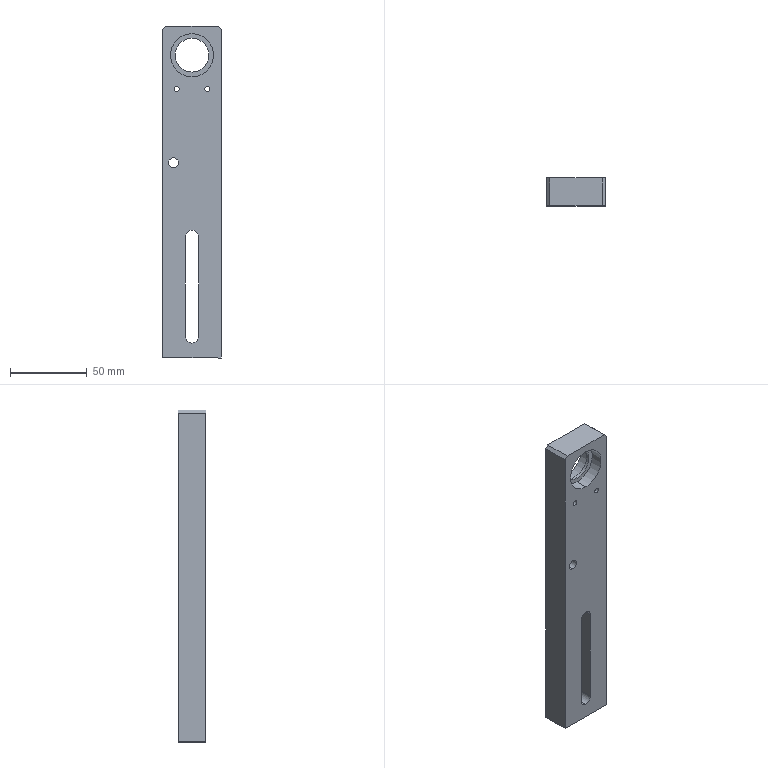Component | SolidWorks | FixedBlock2-1 | 1 solid | 30 faces | box 38 x 18 x 216 mm | volume 124786 mm3 | cylinder 17 | plane 13 | commonest cylinder face diameters 3.3 x4 28 x4 8.5 x3 11 x2 6.5 x2 22 x2
build123d program:
from build123d import *

# Parameters (mm, degrees)
SKETCH1_W                                          = 216
SKETCH1_H                                          = 38
BOSS_EXTRUDE1_DEPTH                                = 18
SKETCH3_R                                          = 11
CUT_EXTRUDE1_DEPTH                                 = 18
SKETCH4_R                                          = 14
CUT_EXTRUDE2_DEPTH                                 = 8
CUT_EXTRUDE3_START                                 = -8
SKETCH5_R                                          = 14
CUT_EXTRUDE3_DEPTH                                 = 8
CUT_EXTRUDE4_DEPTH                                 = 73
CHAMFER1_SIZE                                      = 2
M4_TAPPED_HOLE1_D                                  = 3.3
HOLE_SIZE_ACCORDING_TO_TYPE_1_OF_HEXAG_D           = 6.5
HOLE_SIZE_ACCORDING_TO_TYPE_1_OF_HEXAG_CBORE_D     = 11
HOLE_SIZE_ACCORDING_TO_TYPE_1_OF_HEXAG_CBORE_DEPTH = 6.5


with BuildPart() as part:
    # Sketch1 → Boss-Extrude1 (new body)
    with BuildSketch(Plane.XY):
        Rectangle(SKETCH1_W, SKETCH1_H)
    extrude(amount=BOSS_EXTRUDE1_DEPTH)

    # Sketch3 → Cut-Extrude1 (cut)
    with BuildSketch(Plane.XY.offset(18)):
        with Locations((89, 0)):
            Circle(SKETCH3_R)
    extrude(amount=-CUT_EXTRUDE1_DEPTH, mode=Mode.SUBTRACT)

    # Sketch4 → Cut-Extrude2 (cut)
    with BuildSketch(Plane.XY.offset(18)):
        with Locations((89, 0)):
            Circle(SKETCH4_R)
    extrude(amount=-CUT_EXTRUDE2_DEPTH, mode=Mode.SUBTRACT)

    # Sketch5 → Cut-Extrude3 (cut)
    with BuildSketch(Plane(origin=(0, 0, 0), x_dir=(-1, 0, 0), z_dir=(0, 0, -1)).offset(CUT_EXTRUDE3_START)):
        with Locations(Location((-89, 0, 0), (0, 0, 180))):
            Circle(SKETCH5_R)
    extrude(amount=CUT_EXTRUDE3_DEPTH, mode=Mode.SUBTRACT)

    # Sketch6 → Cut-Extrude4 (cut)
    with BuildSketch(Plane(origin=(0, 0, 0), x_dir=(-1, 0, 0), z_dir=(0, 0, -1))):
        with BuildLine():
            Line((29, 4.25), (94, 4.25))
            ThreePointArc((94, 4.25), (98.25, 0), (94, -4.25))
            Line((94, -4.25), (29, -4.25))
            ThreePointArc((29, -4.25), (24.75, 0), (29, 4.25))
        make_face()
    extrude(amount=-CUT_EXTRUDE4_DEPTH, mode=Mode.SUBTRACT)

    # Chamfer1
    chamfer1_edges = [part.edges().sort_by_distance(p)[0] for p in [
        (108, -19, 9),
        (108, 19, 9),
    ]]
    chamfer(chamfer1_edges, length=CHAMFER1_SIZE)

    # M4 Tapped Hole1 (through all)
    with Locations(Plane(origin=(67, -10, 0), x_dir=(-1, 0, 0), z_dir=(0, 0, -1))):
        with Locations((0, 0), (0, 20)):
            Hole(M4_TAPPED_HOLE1_D / 2)

    # Hole Size _according to_ Type 1 of Hexag (through all)
    with Locations(Plane(origin=(19, -12, 18), x_dir=(1, 0, 0), z_dir=(0, 0, 1))):
        with Locations((0, 0)):
            CounterBoreHole(HOLE_SIZE_ACCORDING_TO_TYPE_1_OF_HEXAG_D / 2, HOLE_SIZE_ACCORDING_TO_TYPE_1_OF_HEXAG_CBORE_D / 2, HOLE_SIZE_ACCORDING_TO_TYPE_1_OF_HEXAG_CBORE_DEPTH)


solid = part.part

# Placed as in the assembly
solid = solid.moved(Location((-48.547, -21.54, 239), (-90, 0, -90)))
STEP:
#1=CARTESIAN_POINT('',(-2.384,-0.3953,9.941));
#2=VERTEX_POINT('',#1);
#3=CARTESIAN_POINT('',(-2.384,-0.3953,10.374));
#4=VERTEX_POINT('',#3);
#5=CARTESIAN_POINT('',(-2.384,-0.3953,10.157));
#6=DIRECTION('',(-0.,1.,-0.));
#7=DIRECTION('',(0.,0.,1.));
#8=AXIS2_PLACEMENT_3D('',#5,#6,#7);
#9=CIRCLE('',#8,0.2165);
#10=EDGE_CURVE('',#2,#4,#9,.T.);
#11=ORIENTED_EDGE('',*,*,#10,.F.);
#12=CARTESIAN_POINT('',(-2.384,-0.1394,9.941));
#13=VERTEX_POINT('',#12);
#14=CARTESIAN_POINT('',(-2.384,-0.1394,9.941));
#15=DIRECTION('',(-0.,1.,-0.));
#16=VECTOR('',#15,39.37);
#17=LINE('',#14,#16);
#18=EDGE_CURVE('',#2,#13,#17,.T.);
#19=ORIENTED_EDGE('',*,*,#18,.T.);
#20=CARTESIAN_POINT('',(-2.384,-0.1394,10.374));
#21=VERTEX_POINT('',#20);
#22=CARTESIAN_POINT('',(-2.384,-0.1394,10.157));
#23=DIRECTION('',(-0.,1.,-0.));
#24=DIRECTION('',(0.,0.,1.));
#25=AXIS2_PLACEMENT_3D('',#22,#23,#24);
#26=CIRCLE('',#25,0.2165);
#27=EDGE_CURVE('',#13,#21,#26,.T.);
#28=ORIENTED_EDGE('',*,*,#27,.T.);
#29=CARTESIAN_POINT('',(-2.384,-0.1394,10.374));
#30=DIRECTION('',(-0.,1.,-0.));
#31=VECTOR('',#30,39.37);
#32=LINE('',#29,#31);
#33=EDGE_CURVE('',#4,#21,#32,.T.);
#34=ORIENTED_EDGE('',*,*,#33,.F.);
#35=EDGE_LOOP('',(#11,#19,#28,#34));
#36=FACE_OUTER_BOUND('',#35,.T.);
#37=CARTESIAN_POINT('',(-2.384,-0.1394,10.157));
#38=DIRECTION('',(-0.,1.,-0.));
#39=DIRECTION('',(0.,0.,1.));
#40=AXIS2_PLACEMENT_3D('',#37,#38,#39);
#41=CYLINDRICAL_SURFACE('',#40,0.2165);
#42=ADVANCED_FACE('',(#36),#41,.F.);
#43=CARTESIAN_POINT('',(-2.384,-0.848,10.285));
#44=VERTEX_POINT('',#43);
#45=CARTESIAN_POINT('',(-2.384,-0.848,10.03));
#46=VERTEX_POINT('',#45);
#47=CARTESIAN_POINT('',(-2.384,-0.848,10.157));
#48=DIRECTION('',(0.,-1.,0.));
#49=DIRECTION('',(-0.,0.,-1.));
#50=AXIS2_PLACEMENT_3D('',#47,#48,#49);
#51=CIRCLE('',#50,0.128);
#52=EDGE_CURVE('',#44,#46,#51,.T.);
#53=ORIENTED_EDGE('',*,*,#52,.T.);
#54=CARTESIAN_POINT('',(-2.384,-0.3953,10.03));
#55=VERTEX_POINT('',#54);
#56=CARTESIAN_POINT('',(-2.384,-0.1394,10.03));
#57=DIRECTION('',(-0.,1.,-0.));
#58=VECTOR('',#57,39.37);
#59=LINE('',#56,#58);
#60=EDGE_CURVE('',#46,#55,#59,.T.);
#61=ORIENTED_EDGE('',*,*,#60,.T.);
#62=CARTESIAN_POINT('',(-2.384,-0.3953,10.285));
#63=VERTEX_POINT('',#62);
#64=CARTESIAN_POINT('',(-2.384,-0.3953,10.157));
#65=DIRECTION('',(-0.,1.,-0.));
#66=DIRECTION('',(0.,0.,1.));
#67=AXIS2_PLACEMENT_3D('',#64,#65,#66);
#68=CIRCLE('',#67,0.128);
#69=EDGE_CURVE('',#55,#63,#68,.T.);
#70=ORIENTED_EDGE('',*,*,#69,.T.);
#71=CARTESIAN_POINT('',(-2.384,-0.1394,10.285));
#72=DIRECTION('',(-0.,1.,-0.));
#73=VECTOR('',#72,39.37);
#74=LINE('',#71,#73);
#75=EDGE_CURVE('',#44,#63,#74,.T.);
#76=ORIENTED_EDGE('',*,*,#75,.F.);
#77=EDGE_LOOP('',(#53,#61,#70,#76));
#78=FACE_OUTER_BOUND('',#77,.T.);
#79=CARTESIAN_POINT('',(-2.384,-0.1394,10.157));
#80=DIRECTION('',(-0.,1.,-0.));
#81=DIRECTION('',(0.,0.,1.));
#82=AXIS2_PLACEMENT_3D('',#79,#80,#81);
#83=CYLINDRICAL_SURFACE('',#82,0.128);
#84=ADVANCED_FACE('',(#78),#83,.F.);
#85=CARTESIAN_POINT('',(-2.305,-0.1394,12.112));
#86=VERTEX_POINT('',#85);
#87=CARTESIAN_POINT('',(-2.305,-0.1394,11.982));
#88=VERTEX_POINT('',#87);
#89=CARTESIAN_POINT('',(-2.305,-0.1394,12.047));
#90=DIRECTION('',(0.,-1.,0.));
#91=DIRECTION('',(-0.,0.,-1.));
#92=AXIS2_PLACEMENT_3D('',#89,#90,#91);
#93=CIRCLE('',#92,0.06496);
#94=EDGE_CURVE('',#86,#88,#93,.T.);
#95=ORIENTED_EDGE('',*,*,#94,.F.);
#96=CARTESIAN_POINT('',(-2.305,-0.848,12.112));
#97=VERTEX_POINT('',#96);
#98=CARTESIAN_POINT('',(-2.305,-0.848,12.112));
#99=DIRECTION('',(0.,-1.,0.));
#100=VECTOR('',#99,39.37);
#101=LINE('',#98,#100);
#102=EDGE_CURVE('',#86,#97,#101,.T.);
#103=ORIENTED_EDGE('',*,*,#102,.T.);
#104=CARTESIAN_POINT('',(-2.305,-0.848,11.982));
#105=VERTEX_POINT('',#104);
#106=CARTESIAN_POINT('',(-2.305,-0.848,12.047));
#107=DIRECTION('',(0.,-1.,0.));
#108=DIRECTION('',(-0.,0.,-1.));
#109=AXIS2_PLACEMENT_3D('',#106,#107,#108);
#110=CIRCLE('',#109,0.06496);
#111=EDGE_CURVE('',#97,#105,#110,.T.);
#112=ORIENTED_EDGE('',*,*,#111,.T.);
#113=CARTESIAN_POINT('',(-2.305,-0.848,11.982));
#114=DIRECTION('',(0.,-1.,0.));
#115=VECTOR('',#114,39.37);
#116=LINE('',#113,#115);
#117=EDGE_CURVE('',#88,#105,#116,.T.);
#118=ORIENTED_EDGE('',*,*,#117,.F.);
#119=EDGE_LOOP('',(#95,#103,#112,#118));
#120=FACE_OUTER_BOUND('',#119,.T.);
#121=CARTESIAN_POINT('',(-2.305,-0.848,12.047));
#122=DIRECTION('',(0.,-1.,0.));
#123=DIRECTION('',(-0.,0.,-1.));
#124=AXIS2_PLACEMENT_3D('',#121,#122,#123);
#125=CYLINDRICAL_SURFACE('',#124,0.06496);
#126=ADVANCED_FACE('',(#120),#125,.F.);
#127=CARTESIAN_POINT('',(-1.518,-0.1394,12.112));
#128=VERTEX_POINT('',#127);
#129=CARTESIAN_POINT('',(-1.518,-0.1394,11.982));
#130=VERTEX_POINT('',#129);
#131=CARTESIAN_POINT('',(-1.518,-0.1394,12.047));
#132=DIRECTION('',(0.,-1.,0.));
#133=DIRECTION('',(-0.,0.,-1.));
#134=AXIS2_PLACEMENT_3D('',#131,#132,#133);
#135=CIRCLE('',#134,0.06496);
#136=EDGE_CURVE('',#128,#130,#135,.T.);
#137=ORIENTED_EDGE('',*,*,#136,.F.);
#138=CARTESIAN_POINT('',(-1.518,-0.848,12.112));
#139=VERTEX_POINT('',#138);
#140=CARTESIAN_POINT('',(-1.518,-0.848,12.112));
#141=DIRECTION('',(0.,-1.,0.));
#142=VECTOR('',#141,39.37);
#143=LINE('',#140,#142);
#144=EDGE_CURVE('',#128,#139,#143,.T.);
#145=ORIENTED_EDGE('',*,*,#144,.T.);
#146=CARTESIAN_POINT('',(-1.518,-0.848,11.982));
#147=VERTEX_POINT('',#146);
#148=CARTESIAN_POINT('',(-1.518,-0.848,12.047));
#149=DIRECTION('',(0.,-1.,0.));
#150=DIRECTION('',(-0.,0.,-1.));
#151=AXIS2_PLACEMENT_3D('',#148,#149,#150);
#152=CIRCLE('',#151,0.06496);
#153=EDGE_CURVE('',#139,#147,#152,.T.);
#154=ORIENTED_EDGE('',*,*,#153,.T.);
#155=CARTESIAN_POINT('',(-1.518,-0.848,11.982));
#156=DIRECTION('',(0.,-1.,0.));
#157=VECTOR('',#156,39.37);
#158=LINE('',#155,#157);
#159=EDGE_CURVE('',#130,#147,#158,.T.);
#160=ORIENTED_EDGE('',*,*,#159,.F.);
#161=EDGE_LOOP('',(#137,#145,#154,#160));
#162=FACE_OUTER_BOUND('',#161,.T.);
#163=CARTESIAN_POINT('',(-1.518,-0.848,12.047));
#164=DIRECTION('',(0.,-1.,0.));
#165=DIRECTION('',(-0.,0.,-1.));
#166=AXIS2_PLACEMENT_3D('',#163,#164,#165);
#167=CYLINDRICAL_SURFACE('',#166,0.06496);
#168=ADVANCED_FACE('',(#162),#167,.F.);
#169=CARTESIAN_POINT('',(-1.911,-0.1394,5.541));
#170=VERTEX_POINT('',#169);
#171=CARTESIAN_POINT('',(-1.744,-0.1394,5.709));
#172=VERTEX_POINT('',#171);
#173=CARTESIAN_POINT('',(-1.911,-0.1394,5.709));
#174=DIRECTION('',(0.,-1.,0.));
#175=DIRECTION('',(-0.,0.,-1.));
#176=AXIS2_PLACEMENT_3D('',#173,#174,#175);
#177=CIRCLE('',#176,0.1673);
#178=EDGE_CURVE('',#170,#172,#177,.T.);
#179=ORIENTED_EDGE('',*,*,#178,.F.);
#180=CARTESIAN_POINT('',(-1.911,-0.848,5.541));
#181=VERTEX_POINT('',#180);
#182=CARTESIAN_POINT('',(-1.911,2.026,5.541));
#183=DIRECTION('',(0.,-1.,0.));
#184=VECTOR('',#183,39.37);
#185=LINE('',#182,#184);
#186=EDGE_CURVE('',#170,#181,#185,.T.);
#187=ORIENTED_EDGE('',*,*,#186,.T.);
#188=CARTESIAN_POINT('',(-1.744,-0.848,5.709));
#189=VERTEX_POINT('',#188);
#190=CARTESIAN_POINT('',(-1.911,-0.848,5.709));
#191=DIRECTION('',(0.,-1.,0.));
#192=DIRECTION('',(-0.,0.,-1.));
#193=AXIS2_PLACEMENT_3D('',#190,#191,#192);
#194=CIRCLE('',#193,0.1673);
#195=EDGE_CURVE('',#181,#189,#194,.T.);
#196=ORIENTED_EDGE('',*,*,#195,.T.);
#197=CARTESIAN_POINT('',(-1.744,2.026,5.709));
#198=DIRECTION('',(0.,-1.,0.));
#199=VECTOR('',#198,39.37);
#200=LINE('',#197,#199);
#201=EDGE_CURVE('',#172,#189,#200,.T.);
#202=ORIENTED_EDGE('',*,*,#201,.F.);
#203=EDGE_LOOP('',(#179,#187,#196,#202));
#204=FACE_OUTER_BOUND('',#203,.T.);
#205=CARTESIAN_POINT('',(-1.911,2.026,5.709));
#206=DIRECTION('',(0.,-1.,0.));
#207=DIRECTION('',(-0.,0.,-1.));
#208=AXIS2_PLACEMENT_3D('',#205,#206,#207);
#209=CYLINDRICAL_SURFACE('',#208,0.1673);
#210=ADVANCED_FACE('',(#204),#209,.F.);
#211=CARTESIAN_POINT('',(-1.911,-0.5331,13.465));
#212=VERTEX_POINT('',#211);
#213=CARTESIAN_POINT('',(-1.911,-0.5331,12.362));
#214=VERTEX_POINT('',#213);
#215=CARTESIAN_POINT('',(-1.911,-0.5331,12.913));
#216=DIRECTION('',(0.,-1.,0.));
#217=DIRECTION('',(-0.,0.,-1.));
#218=AXIS2_PLACEMENT_3D('',#215,#216,#217);
#219=CIRCLE('',#218,0.5512);
#220=EDGE_CURVE('',#212,#214,#219,.T.);
#221=ORIENTED_EDGE('',*,*,#220,.F.);
#222=CARTESIAN_POINT('',(-1.911,-0.848,13.465));
#223=VERTEX_POINT('',#222);
#224=CARTESIAN_POINT('',(-1.911,-0.5331,13.465));
#225=DIRECTION('',(0.,-1.,0.));
#226=VECTOR('',#225,39.37);
#227=LINE('',#224,#226);
#228=EDGE_CURVE('',#212,#223,#227,.T.);
#229=ORIENTED_EDGE('',*,*,#228,.T.);
#230=CARTESIAN_POINT('',(-1.911,-0.848,12.362));
#231=VERTEX_POINT('',#230);
#232=CARTESIAN_POINT('',(-1.911,-0.848,12.913));
#233=DIRECTION('',(0.,-1.,0.));
#234=DIRECTION('',(-0.,0.,-1.));
#235=AXIS2_PLACEMENT_3D('',#232,#233,#234);
#236=CIRCLE('',#235,0.5512);
#237=EDGE_CURVE('',#223,#231,#236,.T.);
#238=ORIENTED_EDGE('',*,*,#237,.T.);
#239=CARTESIAN_POINT('',(-1.911,-0.5331,12.362));
#240=DIRECTION('',(0.,-1.,0.));
#241=VECTOR('',#240,39.37);
#242=LINE('',#239,#241);
#243=EDGE_CURVE('',#214,#231,#242,.T.);
#244=ORIENTED_EDGE('',*,*,#243,.F.);
#245=EDGE_LOOP('',(#221,#229,#238,#244));
#246=FACE_OUTER_BOUND('',#245,.T.);
#247=CARTESIAN_POINT('',(-1.911,-0.5331,12.913));
#248=DIRECTION('',(0.,-1.,0.));
#249=DIRECTION('',(-0.,0.,-1.));
#250=AXIS2_PLACEMENT_3D('',#247,#248,#249);
#251=CYLINDRICAL_SURFACE('',#250,0.5512);
#252=ADVANCED_FACE('',(#246),#251,.F.);
#253=CARTESIAN_POINT('',(-1.911,-0.4543,12.362));
#254=VERTEX_POINT('',#253);
#255=CARTESIAN_POINT('',(-1.911,-0.4543,13.465));
#256=VERTEX_POINT('',#255);
#257=CARTESIAN_POINT('',(-1.911,-0.4543,12.913));
#258=DIRECTION('',(-0.,1.,-0.));
#259=DIRECTION('',(0.,0.,1.));
#260=AXIS2_PLACEMENT_3D('',#257,#258,#259);
#261=CIRCLE('',#260,0.5512);
#262=EDGE_CURVE('',#254,#256,#261,.T.);
#263=ORIENTED_EDGE('',*,*,#262,.F.);
#264=CARTESIAN_POINT('',(-1.911,-0.1394,12.362));
#265=VERTEX_POINT('',#264);
#266=CARTESIAN_POINT('',(-1.911,-0.4543,12.362));
#267=DIRECTION('',(-0.,1.,-0.));
#268=VECTOR('',#267,39.37);
#269=LINE('',#266,#268);
#270=EDGE_CURVE('',#254,#265,#269,.T.);
#271=ORIENTED_EDGE('',*,*,#270,.T.);
#272=CARTESIAN_POINT('',(-1.911,-0.1394,13.465));
#273=VERTEX_POINT('',#272);
#274=CARTESIAN_POINT('',(-1.911,-0.1394,12.913));
#275=DIRECTION('',(-0.,1.,-0.));
#276=DIRECTION('',(0.,0.,1.));
#277=AXIS2_PLACEMENT_3D('',#274,#275,#276);
#278=CIRCLE('',#277,0.5512);
#279=EDGE_CURVE('',#265,#273,#278,.T.);
#280=ORIENTED_EDGE('',*,*,#279,.T.);
#281=CARTESIAN_POINT('',(-1.911,-0.4543,13.465));
#282=DIRECTION('',(-0.,1.,-0.));
#283=VECTOR('',#282,39.37);
#284=LINE('',#281,#283);
#285=EDGE_CURVE('',#256,#273,#284,.T.);
#286=ORIENTED_EDGE('',*,*,#285,.F.);
#287=EDGE_LOOP('',(#263,#271,#280,#286));
#288=FACE_OUTER_BOUND('',#287,.T.);
#289=CARTESIAN_POINT('',(-1.911,-0.4543,12.913));
#290=DIRECTION('',(-0.,1.,-0.));
#291=DIRECTION('',(0.,0.,1.));
#292=AXIS2_PLACEMENT_3D('',#289,#290,#291);
#293=CYLINDRICAL_SURFACE('',#292,0.5512);
#294=ADVANCED_FACE('',(#288),#293,.F.);
#295=CARTESIAN_POINT('',(-1.911,-0.5331,12.48));
#296=VERTEX_POINT('',#295);
#297=CARTESIAN_POINT('',(-1.911,-0.5331,13.346));
#298=VERTEX_POINT('',#297);
#299=CARTESIAN_POINT('',(-1.911,-0.5331,12.913));
#300=DIRECTION('',(-0.,1.,-0.));
#301=DIRECTION('',(-0.,0.,-1.));
#302=AXIS2_PLACEMENT_3D('',#299,#300,#301);
#303=CIRCLE('',#302,0.4331);
#304=EDGE_CURVE('',#296,#298,#303,.T.);
#305=ORIENTED_EDGE('',*,*,#304,.F.);
#306=CARTESIAN_POINT('',(-1.911,-0.4543,12.48));
#307=VERTEX_POINT('',#306);
#308=CARTESIAN_POINT('',(-1.911,-0.848,12.48));
#309=DIRECTION('',(-0.,1.,-0.));
#310=VECTOR('',#309,39.37);
#311=LINE('',#308,#310);
#312=EDGE_CURVE('',#296,#307,#311,.T.);
#313=ORIENTED_EDGE('',*,*,#312,.T.);
#314=CARTESIAN_POINT('',(-1.911,-0.4543,13.346));
#315=VERTEX_POINT('',#314);
#316=CARTESIAN_POINT('',(-1.911,-0.4543,12.913));
#317=DIRECTION('',(0.,-1.,0.));
#318=DIRECTION('',(0.,0.,1.));
#319=AXIS2_PLACEMENT_3D('',#316,#317,#318);
#320=CIRCLE('',#319,0.4331);
#321=EDGE_CURVE('',#315,#307,#320,.T.);
#322=ORIENTED_EDGE('',*,*,#321,.F.);
#323=CARTESIAN_POINT('',(-1.911,-0.848,13.346));
#324=DIRECTION('',(-0.,1.,-0.));
#325=VECTOR('',#324,39.37);
#326=LINE('',#323,#325);
#327=EDGE_CURVE('',#298,#315,#326,.T.);
#328=ORIENTED_EDGE('',*,*,#327,.F.);
#329=EDGE_LOOP('',(#305,#313,#322,#328));
#330=FACE_OUTER_BOUND('',#329,.T.);
#331=CARTESIAN_POINT('',(-1.911,-0.848,12.913));
#332=DIRECTION('',(-0.,1.,-0.));
#333=DIRECTION('',(0.,0.,1.));
#334=AXIS2_PLACEMENT_3D('',#331,#332,#333);
#335=CYLINDRICAL_SURFACE('',#334,0.4331);
#336=ADVANCED_FACE('',(#330),#335,.F.);
#337=CARTESIAN_POINT('',(-2.305,-0.1394,12.047));
#338=DIRECTION('',(0.,-1.,0.));
#339=DIRECTION('',(-0.,0.,-1.));
#340=AXIS2_PLACEMENT_3D('',#337,#338,#339);
#341=CIRCLE('',#340,0.06496);
#342=EDGE_CURVE('',#88,#86,#341,.T.);
#343=ORIENTED_EDGE('',*,*,#342,.T.);
#344=ORIENTED_EDGE('',*,*,#94,.T.);
#345=EDGE_LOOP('',(#343,#344));
#346=FACE_BOUND('',#345,.T.);
#347=CARTESIAN_POINT('',(-1.518,-0.1394,12.047));
#348=DIRECTION('',(0.,-1.,0.));
#349=DIRECTION('',(-0.,0.,-1.));
#350=AXIS2_PLACEMENT_3D('',#347,#348,#349);
#351=CIRCLE('',#350,0.06496);
#352=EDGE_CURVE('',#130,#128,#351,.T.);
#353=ORIENTED_EDGE('',*,*,#352,.T.);
#354=ORIENTED_EDGE('',*,*,#136,.T.);
#355=EDGE_LOOP('',(#353,#354));
#356=FACE_BOUND('',#355,.T.);
#357=CARTESIAN_POINT('',(-1.744,-0.1394,8.268));
#358=VERTEX_POINT('',#357);
#359=CARTESIAN_POINT('',(-1.744,-0.1394,9.409));
#360=DIRECTION('',(0.,0.,1.));
#361=VECTOR('',#360,39.37);
#362=LINE('',#359,#361);
#363=EDGE_CURVE('',#172,#358,#362,.T.);
#364=ORIENTED_EDGE('',*,*,#363,.T.);
#365=CARTESIAN_POINT('',(-2.079,-0.1394,8.268));
#366=VERTEX_POINT('',#365);
#367=CARTESIAN_POINT('',(-1.911,-0.1394,8.268));
#368=DIRECTION('',(0.,-1.,0.));
#369=DIRECTION('',(-0.,0.,-1.));
#370=AXIS2_PLACEMENT_3D('',#367,#368,#369);
#371=CIRCLE('',#370,0.1673);
#372=EDGE_CURVE('',#358,#366,#371,.T.);
#373=ORIENTED_EDGE('',*,*,#372,.T.);
#374=CARTESIAN_POINT('',(-2.079,-0.1394,5.709));
#375=VERTEX_POINT('',#374);
#376=CARTESIAN_POINT('',(-2.079,-0.1394,9.409));
#377=DIRECTION('',(-0.,-0.,-1.));
#378=VECTOR('',#377,39.37);
#379=LINE('',#376,#378);
#380=EDGE_CURVE('',#366,#375,#379,.T.);
#381=ORIENTED_EDGE('',*,*,#380,.T.);
#382=CARTESIAN_POINT('',(-1.911,-0.1394,5.709));
#383=DIRECTION('',(0.,-1.,0.));
#384=DIRECTION('',(-0.,0.,-1.));
#385=AXIS2_PLACEMENT_3D('',#382,#383,#384);
#386=CIRCLE('',#385,0.1673);
#387=EDGE_CURVE('',#375,#170,#386,.T.);
#388=ORIENTED_EDGE('',*,*,#387,.T.);
#389=ORIENTED_EDGE('',*,*,#178,.T.);
#390=EDGE_LOOP('',(#364,#373,#381,#388,#389));
#391=FACE_BOUND('',#390,.T.);
#392=CARTESIAN_POINT('',(-1.911,-0.1394,12.913));
#393=DIRECTION('',(-0.,1.,-0.));
#394=DIRECTION('',(0.,0.,1.));
#395=AXIS2_PLACEMENT_3D('',#392,#393,#394);
#396=CIRCLE('',#395,0.5512);
#397=EDGE_CURVE('',#273,#265,#396,.T.);
#398=ORIENTED_EDGE('',*,*,#397,.F.);
#399=ORIENTED_EDGE('',*,*,#279,.F.);
#400=EDGE_LOOP('',(#398,#399));
#401=FACE_BOUND('',#400,.T.);
#402=CARTESIAN_POINT('',(-2.659,-0.1394,5.157));
#403=VERTEX_POINT('',#402);
#404=CARTESIAN_POINT('',(-2.659,-0.1394,13.583));
#405=VERTEX_POINT('',#404);
#406=CARTESIAN_POINT('',(-2.659,-0.1394,5.157));
#407=DIRECTION('',(0.,0.,1.));
#408=VECTOR('',#407,39.37);
#409=LINE('',#406,#408);
#410=EDGE_CURVE('',#403,#405,#409,.T.);
#411=ORIENTED_EDGE('',*,*,#410,.T.);
#412=CARTESIAN_POINT('',(-2.581,-0.1394,13.661));
#413=VERTEX_POINT('',#412);
#414=CARTESIAN_POINT('',(-2.581,-0.1394,13.661));
#415=DIRECTION('',(0.7071,0.,0.7071));
#416=VECTOR('',#415,39.37);
#417=LINE('',#414,#416);
#418=EDGE_CURVE('',#405,#413,#417,.T.);
#419=ORIENTED_EDGE('',*,*,#418,.T.);
#420=CARTESIAN_POINT('',(-1.242,-0.1394,13.661));
#421=VERTEX_POINT('',#420);
#422=CARTESIAN_POINT('',(-2.659,-0.1394,13.661));
#423=DIRECTION('',(1.,0.,-0.));
#424=VECTOR('',#423,39.37);
#425=LINE('',#422,#424);
#426=EDGE_CURVE('',#413,#421,#425,.T.);
#427=ORIENTED_EDGE('',*,*,#426,.T.);
#428=CARTESIAN_POINT('',(-1.163,-0.1394,13.583));
#429=VERTEX_POINT('',#428);
#430=CARTESIAN_POINT('',(-1.163,-0.1394,13.583));
#431=DIRECTION('',(0.7071,0.,-0.7071));
#432=VECTOR('',#431,39.37);
#433=LINE('',#430,#432);
#434=EDGE_CURVE('',#421,#429,#433,.T.);
#435=ORIENTED_EDGE('',*,*,#434,.T.);
#436=CARTESIAN_POINT('',(-1.163,-0.1394,5.157));
#437=VERTEX_POINT('',#436);
#438=CARTESIAN_POINT('',(-1.163,-0.1394,5.157));
#439=DIRECTION('',(-0.,-0.,-1.));
#440=VECTOR('',#439,39.37);
#441=LINE('',#438,#440);
#442=EDGE_CURVE('',#429,#437,#441,.T.);
#443=ORIENTED_EDGE('',*,*,#442,.T.);
#444=CARTESIAN_POINT('',(-2.659,-0.1394,5.157));
#445=DIRECTION('',(-1.,-0.,0.));
#446=VECTOR('',#445,39.37);
#447=LINE('',#444,#446);
#448=EDGE_CURVE('',#437,#403,#447,.T.);
#449=ORIENTED_EDGE('',*,*,#448,.T.);
#450=EDGE_LOOP('',(#411,#419,#427,#435,#443,#449));
#451=FACE_OUTER_BOUND('',#450,.T.);
#452=CARTESIAN_POINT('',(-2.384,-0.1394,10.157));
#453=DIRECTION('',(-0.,1.,-0.));
#454=DIRECTION('',(0.,0.,1.));
#455=AXIS2_PLACEMENT_3D('',#452,#453,#454);
#456=CIRCLE('',#455,0.2165);
#457=EDGE_CURVE('',#21,#13,#456,.T.);
#458=ORIENTED_EDGE('',*,*,#457,.F.);
#459=ORIENTED_EDGE('',*,*,#27,.F.);
#460=EDGE_LOOP('',(#458,#459));
#461=FACE_BOUND('',#460,.T.);
#462=CARTESIAN_POINT('',(-1.911,-0.1394,9.409));
#463=DIRECTION('',(0.,-1.,0.));
#464=DIRECTION('',(-0.,-0.,-1.));
#465=AXIS2_PLACEMENT_3D('',#462,#463,#464);
#466=PLANE('',#465);
#467=ADVANCED_FACE('',(#346,#356,#391,#401,#451,#461),#466,.F.);
#468=ORIENTED_EDGE('',*,*,#312,.F.);
#469=CARTESIAN_POINT('',(-1.911,-0.5331,12.913));
#470=DIRECTION('',(-0.,1.,-0.));
#471=DIRECTION('',(-0.,0.,-1.));
#472=AXIS2_PLACEMENT_3D('',#469,#470,#471);
#473=CIRCLE('',#472,0.4331);
#474=EDGE_CURVE('',#298,#296,#473,.T.);
#475=ORIENTED_EDGE('',*,*,#474,.F.);
#476=ORIENTED_EDGE('',*,*,#327,.T.);
#477=CARTESIAN_POINT('',(-1.911,-0.4543,12.913));
#478=DIRECTION('',(0.,-1.,0.));
#479=DIRECTION('',(0.,0.,1.));
#480=AXIS2_PLACEMENT_3D('',#477,#478,#479);
#481=CIRCLE('',#480,0.4331);
#482=EDGE_CURVE('',#307,#315,#481,.T.);
#483=ORIENTED_EDGE('',*,*,#482,.F.);
#484=EDGE_LOOP('',(#468,#475,#476,#483));
#485=FACE_OUTER_BOUND('',#484,.T.);
#486=CARTESIAN_POINT('',(-1.911,-0.848,12.913));
#487=DIRECTION('',(-0.,1.,-0.));
#488=DIRECTION('',(0.,0.,1.));
#489=AXIS2_PLACEMENT_3D('',#486,#487,#488);
#490=CYLINDRICAL_SURFACE('',#489,0.4331);
#491=ADVANCED_FACE('',(#485),#490,.F.);
#492=ORIENTED_EDGE('',*,*,#426,.F.);
#493=CARTESIAN_POINT('',(-2.581,-0.848,13.661));
#494=VERTEX_POINT('',#493);
#495=CARTESIAN_POINT('',(-2.581,-0.1394,13.661));
#496=DIRECTION('',(0.,-1.,0.));
#497=VECTOR('',#496,39.37);
#498=LINE('',#495,#497);
#499=EDGE_CURVE('',#413,#494,#498,.T.);
#500=ORIENTED_EDGE('',*,*,#499,.T.);
#501=CARTESIAN_POINT('',(-1.242,-0.848,13.661));
#502=VERTEX_POINT('',#501);
#503=CARTESIAN_POINT('',(-2.659,-0.848,13.661));
#504=DIRECTION('',(1.,0.,-0.));
#505=VECTOR('',#504,39.37);
#506=LINE('',#503,#505);
#507=EDGE_CURVE('',#494,#502,#506,.T.);
#508=ORIENTED_EDGE('',*,*,#507,.T.);
#509=CARTESIAN_POINT('',(-1.242,-0.1394,13.661));
#510=DIRECTION('',(-0.,1.,-0.));
#511=VECTOR('',#510,39.37);
#512=LINE('',#509,#511);
#513=EDGE_CURVE('',#502,#421,#512,.T.);
#514=ORIENTED_EDGE('',*,*,#513,.T.);
#515=EDGE_LOOP('',(#492,#500,#508,#514));
#516=FACE_OUTER_BOUND('',#515,.T.);
#517=CARTESIAN_POINT('',(-2.659,-0.1394,13.661));
#518=DIRECTION('',(-0.,-0.,-1.));
#519=DIRECTION('',(-0.,1.,-0.));
#520=AXIS2_PLACEMENT_3D('',#517,#518,#519);
#521=PLANE('',#520);
#522=ADVANCED_FACE('',(#516),#521,.F.);
#523=ORIENTED_EDGE('',*,*,#442,.F.);
#524=CARTESIAN_POINT('',(-1.163,-0.848,13.583));
#525=VERTEX_POINT('',#524);
#526=CARTESIAN_POINT('',(-1.163,-0.1394,13.583));
#527=DIRECTION('',(0.,-1.,0.));
#528=VECTOR('',#527,39.37);
#529=LINE('',#526,#528);
#530=EDGE_CURVE('',#429,#525,#529,.T.);
#531=ORIENTED_EDGE('',*,*,#530,.T.);
#532=CARTESIAN_POINT('',(-1.163,-0.848,5.157));
#533=VERTEX_POINT('',#532);
#534=CARTESIAN_POINT('',(-1.163,-0.848,5.157));
#535=DIRECTION('',(-0.,-0.,-1.));
#536=VECTOR('',#535,39.37);
#537=LINE('',#534,#536);
#538=EDGE_CURVE('',#525,#533,#537,.T.);
#539=ORIENTED_EDGE('',*,*,#538,.T.);
#540=CARTESIAN_POINT('',(-1.163,-0.1394,5.157));
#541=DIRECTION('',(0.,-1.,0.));
#542=VECTOR('',#541,39.37);
#543=LINE('',#540,#542);
#544=EDGE_CURVE('',#437,#533,#543,.T.);
#545=ORIENTED_EDGE('',*,*,#544,.F.);
#546=EDGE_LOOP('',(#523,#531,#539,#545));
#547=FACE_OUTER_BOUND('',#546,.T.);
#548=CARTESIAN_POINT('',(-1.163,-0.1394,5.157));
#549=DIRECTION('',(-1.,-0.,0.));
#550=DIRECTION('',(0.,-1.,0.));
#551=AXIS2_PLACEMENT_3D('',#548,#549,#550);
#552=PLANE('',#551);
#553=ADVANCED_FACE('',(#547),#552,.F.);
#554=CARTESIAN_POINT('',(-2.659,-0.848,5.157));
#555=VERTEX_POINT('',#554);
#556=CARTESIAN_POINT('',(-2.659,-0.848,5.157));
#557=DIRECTION('',(-1.,-0.,0.));
#558=VECTOR('',#557,39.37);
#559=LINE('',#556,#558);
#560=EDGE_CURVE('',#533,#555,#559,.T.);
#561=ORIENTED_EDGE('',*,*,#560,.T.);
#562=CARTESIAN_POINT('',(-2.659,-0.1394,5.157));
#563=DIRECTION('',(0.,-1.,0.));
#564=VECTOR('',#563,39.37);
#565=LINE('',#562,#564);
#566=EDGE_CURVE('',#403,#555,#565,.T.);
#567=ORIENTED_EDGE('',*,*,#566,.F.);
#568=ORIENTED_EDGE('',*,*,#448,.F.);
#569=ORIENTED_EDGE('',*,*,#544,.T.);
#570=EDGE_LOOP('',(#561,#567,#568,#569));
#571=FACE_OUTER_BOUND('',#570,.T.);
#572=CARTESIAN_POINT('',(-2.659,-0.1394,5.157));
#573=DIRECTION('',(0.,0.,1.));
#574=DIRECTION('',(0.,-1.,0.));
#575=AXIS2_PLACEMENT_3D('',#572,#573,#574);
#576=PLANE('',#575);
#577=ADVANCED_FACE('',(#571),#576,.F.);
#578=CARTESIAN_POINT('',(-2.659,-0.848,13.583));
#579=VERTEX_POINT('',#578);
#580=CARTESIAN_POINT('',(-2.659,-0.848,5.157));
#581=DIRECTION('',(0.,0.,1.));
#582=VECTOR('',#581,39.37);
#583=LINE('',#580,#582);
#584=EDGE_CURVE('',#555,#579,#583,.T.);
#585=ORIENTED_EDGE('',*,*,#584,.T.);
#586=CARTESIAN_POINT('',(-2.659,-0.1394,13.583));
#587=DIRECTION('',(-0.,1.,-0.));
#588=VECTOR('',#587,39.37);
#589=LINE('',#586,#588);
#590=EDGE_CURVE('',#579,#405,#589,.T.);
#591=ORIENTED_EDGE('',*,*,#590,.T.);
#592=ORIENTED_EDGE('',*,*,#410,.F.);
#593=ORIENTED_EDGE('',*,*,#566,.T.);
#594=EDGE_LOOP('',(#585,#591,#592,#593));
#595=FACE_OUTER_BOUND('',#594,.T.);
#596=CARTESIAN_POINT('',(-2.659,-0.1394,5.157));
#597=DIRECTION('',(1.,0.,-0.));
#598=DIRECTION('',(-0.,1.,-0.));
#599=AXIS2_PLACEMENT_3D('',#596,#597,#598);
#600=PLANE('',#599);
#601=ADVANCED_FACE('',(#595),#600,.F.);
#602=ORIENTED_EDGE('',*,*,#52,.F.);
#603=CARTESIAN_POINT('',(-2.384,-0.848,10.157));
#604=DIRECTION('',(0.,-1.,0.));
#605=DIRECTION('',(-0.,0.,-1.));
#606=AXIS2_PLACEMENT_3D('',#603,#604,#605);
#607=CIRCLE('',#606,0.128);
#608=EDGE_CURVE('',#46,#44,#607,.T.);
#609=ORIENTED_EDGE('',*,*,#608,.F.);
#610=EDGE_LOOP('',(#602,#609));
#611=FACE_BOUND('',#610,.T.);
#612=CARTESIAN_POINT('',(-2.305,-0.848,12.047));
#613=DIRECTION('',(0.,-1.,0.));
#614=DIRECTION('',(-0.,0.,-1.));
#615=AXIS2_PLACEMENT_3D('',#612,#613,#614);
#616=CIRCLE('',#615,0.06496);
#617=EDGE_CURVE('',#105,#97,#616,.T.);
#618=ORIENTED_EDGE('',*,*,#617,.F.);
#619=ORIENTED_EDGE('',*,*,#111,.F.);
#620=EDGE_LOOP('',(#618,#619));
#621=FACE_BOUND('',#620,.T.);
#622=CARTESIAN_POINT('',(-1.518,-0.848,12.047));
#623=DIRECTION('',(0.,-1.,0.));
#624=DIRECTION('',(-0.,0.,-1.));
#625=AXIS2_PLACEMENT_3D('',#622,#623,#624);
#626=CIRCLE('',#625,0.06496);
#627=EDGE_CURVE('',#147,#139,#626,.T.);
#628=ORIENTED_EDGE('',*,*,#627,.F.);
#629=ORIENTED_EDGE('',*,*,#153,.F.);
#630=EDGE_LOOP('',(#628,#629));
#631=FACE_BOUND('',#630,.T.);
#632=CARTESIAN_POINT('',(-1.744,-0.848,8.268));
#633=VERTEX_POINT('',#632);
#634=CARTESIAN_POINT('',(-2.079,-0.848,8.268));
#635=VERTEX_POINT('',#634);
#636=CARTESIAN_POINT('',(-1.911,-0.848,8.268));
#637=DIRECTION('',(0.,-1.,0.));
#638=DIRECTION('',(-0.,0.,-1.));
#639=AXIS2_PLACEMENT_3D('',#636,#637,#638);
#640=CIRCLE('',#639,0.1673);
#641=EDGE_CURVE('',#633,#635,#640,.T.);
#642=ORIENTED_EDGE('',*,*,#641,.F.);
#643=CARTESIAN_POINT('',(-1.744,-0.848,8.268));
#644=DIRECTION('',(0.,0.,1.));
#645=VECTOR('',#644,39.37);
#646=LINE('',#643,#645);
#647=EDGE_CURVE('',#189,#633,#646,.T.);
#648=ORIENTED_EDGE('',*,*,#647,.F.);
#649=ORIENTED_EDGE('',*,*,#195,.F.);
#650=CARTESIAN_POINT('',(-2.079,-0.848,5.709));
#651=VERTEX_POINT('',#650);
#652=CARTESIAN_POINT('',(-1.911,-0.848,5.709));
#653=DIRECTION('',(0.,-1.,0.));
#654=DIRECTION('',(-0.,0.,-1.));
#655=AXIS2_PLACEMENT_3D('',#652,#653,#654);
#656=CIRCLE('',#655,0.1673);
#657=EDGE_CURVE('',#651,#181,#656,.T.);
#658=ORIENTED_EDGE('',*,*,#657,.F.);
#659=CARTESIAN_POINT('',(-2.079,-0.848,8.268));
#660=DIRECTION('',(-0.,-0.,-1.));
#661=VECTOR('',#660,39.37);
#662=LINE('',#659,#661);
#663=EDGE_CURVE('',#635,#651,#662,.T.);
#664=ORIENTED_EDGE('',*,*,#663,.F.);
#665=EDGE_LOOP('',(#642,#648,#649,#658,#664));
#666=FACE_BOUND('',#665,.T.);
#667=CARTESIAN_POINT('',(-1.911,-0.848,12.913));
#668=DIRECTION('',(0.,-1.,0.));
#669=DIRECTION('',(-0.,0.,-1.));
#670=AXIS2_PLACEMENT_3D('',#667,#668,#669);
#671=CIRCLE('',#670,0.5512);
#672=EDGE_CURVE('',#231,#223,#671,.T.);
#673=ORIENTED_EDGE('',*,*,#672,.F.);
#674=ORIENTED_EDGE('',*,*,#237,.F.);
#675=EDGE_LOOP('',(#673,#674));
#676=FACE_BOUND('',#675,.T.);
#677=ORIENTED_EDGE('',*,*,#507,.F.);
#678=CARTESIAN_POINT('',(-4.372,-0.848,11.87));
#679=DIRECTION('',(-0.7071,-0.,-0.7071));
#680=VECTOR('',#679,39.37);
#681=LINE('',#678,#680);
#682=EDGE_CURVE('',#494,#579,#681,.T.);
#683=ORIENTED_EDGE('',*,*,#682,.T.);
#684=ORIENTED_EDGE('',*,*,#584,.F.);
#685=ORIENTED_EDGE('',*,*,#560,.F.);
#686=ORIENTED_EDGE('',*,*,#538,.F.);
#687=CARTESIAN_POINT('',(0.5493,-0.848,11.87));
#688=DIRECTION('',(-0.7071,-0.,0.7071));
#689=VECTOR('',#688,39.37);
#690=LINE('',#687,#689);
#691=EDGE_CURVE('',#525,#502,#690,.T.);
#692=ORIENTED_EDGE('',*,*,#691,.T.);
#693=EDGE_LOOP('',(#677,#683,#684,#685,#686,#692));
#694=FACE_OUTER_BOUND('',#693,.T.);
#695=CARTESIAN_POINT('',(-1.911,-0.848,9.409));
#696=DIRECTION('',(0.,-1.,0.));
#697=DIRECTION('',(-0.,-0.,-1.));
#698=AXIS2_PLACEMENT_3D('',#695,#696,#697);
#699=PLANE('',#698);
#700=ADVANCED_FACE('',(#611,#621,#631,#666,#676,#694),#699,.T.);
#701=CARTESIAN_POINT('',(-1.911,-0.4543,12.913));
#702=DIRECTION('',(-0.,1.,-0.));
#703=DIRECTION('',(0.,0.,1.));
#704=AXIS2_PLACEMENT_3D('',#701,#702,#703);
#705=CIRCLE('',#704,0.5512);
#706=EDGE_CURVE('',#256,#254,#705,.T.);
#707=ORIENTED_EDGE('',*,*,#706,.T.);
#708=ORIENTED_EDGE('',*,*,#262,.T.);
#709=EDGE_LOOP('',(#707,#708));
#710=FACE_OUTER_BOUND('',#709,.T.);
#711=ORIENTED_EDGE('',*,*,#321,.T.);
#712=ORIENTED_EDGE('',*,*,#482,.T.);
#713=EDGE_LOOP('',(#711,#712));
#714=FACE_BOUND('',#713,.T.);
#715=CARTESIAN_POINT('',(-1.911,-0.4543,12.913));
#716=DIRECTION('',(-0.,1.,-0.));
#717=DIRECTION('',(0.,0.,1.));
#718=AXIS2_PLACEMENT_3D('',#715,#716,#717);
#719=PLANE('',#718);
#720=ADVANCED_FACE('',(#710,#714),#719,.T.);
#721=ORIENTED_EDGE('',*,*,#270,.F.);
#722=ORIENTED_EDGE('',*,*,#706,.F.);
#723=ORIENTED_EDGE('',*,*,#285,.T.);
#724=ORIENTED_EDGE('',*,*,#397,.T.);
#725=EDGE_LOOP('',(#721,#722,#723,#724));
#726=FACE_OUTER_BOUND('',#725,.T.);
#727=CARTESIAN_POINT('',(-1.911,-0.4543,12.913));
#728=DIRECTION('',(-0.,1.,-0.));
#729=DIRECTION('',(0.,0.,1.));
#730=AXIS2_PLACEMENT_3D('',#727,#728,#729);
#731=CYLINDRICAL_SURFACE('',#730,0.5512);
#732=ADVANCED_FACE('',(#726),#731,.F.);
#733=CARTESIAN_POINT('',(-1.911,-0.5331,12.913));
#734=DIRECTION('',(0.,-1.,0.));
#735=DIRECTION('',(-0.,0.,-1.));
#736=AXIS2_PLACEMENT_3D('',#733,#734,#735);
#737=CIRCLE('',#736,0.5512);
#738=EDGE_CURVE('',#214,#212,#737,.T.);
#739=ORIENTED_EDGE('',*,*,#738,.T.);
#740=ORIENTED_EDGE('',*,*,#220,.T.);
#741=EDGE_LOOP('',(#739,#740));
#742=FACE_OUTER_BOUND('',#741,.T.);
#743=ORIENTED_EDGE('',*,*,#474,.T.);
#744=ORIENTED_EDGE('',*,*,#304,.T.);
#745=EDGE_LOOP('',(#743,#744));
#746=FACE_BOUND('',#745,.T.);
#747=CARTESIAN_POINT('',(-1.911,-0.5331,12.913));
#748=DIRECTION('',(0.,-1.,0.));
#749=DIRECTION('',(-0.,-0.,-1.));
#750=AXIS2_PLACEMENT_3D('',#747,#748,#749);
#751=PLANE('',#750);
#752=ADVANCED_FACE('',(#742,#746),#751,.T.);
#753=ORIENTED_EDGE('',*,*,#228,.F.);
#754=ORIENTED_EDGE('',*,*,#738,.F.);
#755=ORIENTED_EDGE('',*,*,#243,.T.);
#756=ORIENTED_EDGE('',*,*,#672,.T.);
#757=EDGE_LOOP('',(#753,#754,#755,#756));
#758=FACE_OUTER_BOUND('',#757,.T.);
#759=CARTESIAN_POINT('',(-1.911,-0.5331,12.913));
#760=DIRECTION('',(0.,-1.,0.));
#761=DIRECTION('',(-0.,0.,-1.));
#762=AXIS2_PLACEMENT_3D('',#759,#760,#761);
#763=CYLINDRICAL_SURFACE('',#762,0.5512);
#764=ADVANCED_FACE('',(#758),#763,.F.);
#765=CARTESIAN_POINT('',(-1.744,2.026,8.268));
#766=DIRECTION('',(0.,-1.,0.));
#767=VECTOR('',#766,39.37);
#768=LINE('',#765,#767);
#769=EDGE_CURVE('',#358,#633,#768,.T.);
#770=ORIENTED_EDGE('',*,*,#769,.T.);
#771=ORIENTED_EDGE('',*,*,#641,.T.);
#772=CARTESIAN_POINT('',(-2.079,2.026,8.268));
#773=DIRECTION('',(0.,-1.,0.));
#774=VECTOR('',#773,39.37);
#775=LINE('',#772,#774);
#776=EDGE_CURVE('',#366,#635,#775,.T.);
#777=ORIENTED_EDGE('',*,*,#776,.F.);
#778=ORIENTED_EDGE('',*,*,#372,.F.);
#779=EDGE_LOOP('',(#770,#771,#777,#778));
#780=FACE_OUTER_BOUND('',#779,.T.);
#781=CARTESIAN_POINT('',(-1.911,2.026,8.268));
#782=DIRECTION('',(0.,-1.,0.));
#783=DIRECTION('',(-0.,0.,-1.));
#784=AXIS2_PLACEMENT_3D('',#781,#782,#783);
#785=CYLINDRICAL_SURFACE('',#784,0.1673);
#786=ADVANCED_FACE('',(#780),#785,.F.);
#787=ORIENTED_EDGE('',*,*,#201,.T.);
#788=ORIENTED_EDGE('',*,*,#647,.T.);
#789=ORIENTED_EDGE('',*,*,#769,.F.);
#790=ORIENTED_EDGE('',*,*,#363,.F.);
#791=EDGE_LOOP('',(#787,#788,#789,#790));
#792=FACE_OUTER_BOUND('',#791,.T.);
#793=CARTESIAN_POINT('',(-1.744,2.026,8.268));
#794=DIRECTION('',(1.,0.,-0.));
#795=DIRECTION('',(-0.,-0.,-1.));
#796=AXIS2_PLACEMENT_3D('',#793,#794,#795);
#797=PLANE('',#796);
#798=ADVANCED_FACE('',(#792),#797,.F.);
#799=ORIENTED_EDGE('',*,*,#186,.F.);
#800=ORIENTED_EDGE('',*,*,#387,.F.);
#801=CARTESIAN_POINT('',(-2.079,2.026,5.709));
#802=DIRECTION('',(0.,-1.,0.));
#803=VECTOR('',#802,39.37);
#804=LINE('',#801,#803);
#805=EDGE_CURVE('',#375,#651,#804,.T.);
#806=ORIENTED_EDGE('',*,*,#805,.T.);
#807=ORIENTED_EDGE('',*,*,#657,.T.);
#808=EDGE_LOOP('',(#799,#800,#806,#807));
#809=FACE_OUTER_BOUND('',#808,.T.);
#810=CARTESIAN_POINT('',(-1.911,2.026,5.709));
#811=DIRECTION('',(0.,-1.,0.));
#812=DIRECTION('',(-0.,0.,-1.));
#813=AXIS2_PLACEMENT_3D('',#810,#811,#812);
#814=CYLINDRICAL_SURFACE('',#813,0.1673);
#815=ADVANCED_FACE('',(#809),#814,.F.);
#816=ORIENTED_EDGE('',*,*,#776,.T.);
#817=ORIENTED_EDGE('',*,*,#663,.T.);
#818=ORIENTED_EDGE('',*,*,#805,.F.);
#819=ORIENTED_EDGE('',*,*,#380,.F.);
#820=EDGE_LOOP('',(#816,#817,#818,#819));
#821=FACE_OUTER_BOUND('',#820,.T.);
#822=CARTESIAN_POINT('',(-2.079,2.026,8.268));
#823=DIRECTION('',(-1.,-0.,0.));
#824=DIRECTION('',(0.,0.,1.));
#825=AXIS2_PLACEMENT_3D('',#822,#823,#824);
#826=PLANE('',#825);
#827=ADVANCED_FACE('',(#821),#826,.F.);
#828=ORIENTED_EDGE('',*,*,#418,.F.);
#829=ORIENTED_EDGE('',*,*,#590,.F.);
#830=ORIENTED_EDGE('',*,*,#682,.F.);
#831=ORIENTED_EDGE('',*,*,#499,.F.);
#832=EDGE_LOOP('',(#828,#829,#830,#831));
#833=FACE_OUTER_BOUND('',#832,.T.);
#834=CARTESIAN_POINT('',(-2.581,-0.1394,13.661));
#835=DIRECTION('',(0.7071,0.,-0.7071));
#836=DIRECTION('',(0.,-1.,0.));
#837=AXIS2_PLACEMENT_3D('',#834,#835,#836);
#838=PLANE('',#837);
#839=ADVANCED_FACE('',(#833),#838,.F.);
#840=ORIENTED_EDGE('',*,*,#434,.F.);
#841=ORIENTED_EDGE('',*,*,#513,.F.);
#842=ORIENTED_EDGE('',*,*,#691,.F.);
#843=ORIENTED_EDGE('',*,*,#530,.F.);
#844=EDGE_LOOP('',(#840,#841,#842,#843));
#845=FACE_OUTER_BOUND('',#844,.T.);
#846=CARTESIAN_POINT('',(-1.163,-0.1394,13.583));
#847=DIRECTION('',(-0.7071,-0.,-0.7071));
#848=DIRECTION('',(0.,-1.,0.));
#849=AXIS2_PLACEMENT_3D('',#846,#847,#848);
#850=PLANE('',#849);
#851=ADVANCED_FACE('',(#845),#850,.F.);
#852=ORIENTED_EDGE('',*,*,#144,.F.);
#853=ORIENTED_EDGE('',*,*,#352,.F.);
#854=ORIENTED_EDGE('',*,*,#159,.T.);
#855=ORIENTED_EDGE('',*,*,#627,.T.);
#856=EDGE_LOOP('',(#852,#853,#854,#855));
#857=FACE_OUTER_BOUND('',#856,.T.);
#858=CARTESIAN_POINT('',(-1.518,-0.848,12.047));
#859=DIRECTION('',(0.,-1.,0.));
#860=DIRECTION('',(-0.,0.,-1.));
#861=AXIS2_PLACEMENT_3D('',#858,#859,#860);
#862=CYLINDRICAL_SURFACE('',#861,0.06496);
#863=ADVANCED_FACE('',(#857),#862,.F.);
#864=ORIENTED_EDGE('',*,*,#102,.F.);
#865=ORIENTED_EDGE('',*,*,#342,.F.);
#866=ORIENTED_EDGE('',*,*,#117,.T.);
#867=ORIENTED_EDGE('',*,*,#617,.T.);
#868=EDGE_LOOP('',(#864,#865,#866,#867));
#869=FACE_OUTER_BOUND('',#868,.T.);
#870=CARTESIAN_POINT('',(-2.305,-0.848,12.047));
#871=DIRECTION('',(0.,-1.,0.));
#872=DIRECTION('',(-0.,0.,-1.));
#873=AXIS2_PLACEMENT_3D('',#870,#871,#872);
#874=CYLINDRICAL_SURFACE('',#873,0.06496);
#875=ADVANCED_FACE('',(#869),#874,.F.);
#876=ORIENTED_EDGE('',*,*,#60,.F.);
#877=ORIENTED_EDGE('',*,*,#608,.T.);
#878=ORIENTED_EDGE('',*,*,#75,.T.);
#879=CARTESIAN_POINT('',(-2.384,-0.3953,10.157));
#880=DIRECTION('',(-0.,1.,-0.));
#881=DIRECTION('',(0.,0.,1.));
#882=AXIS2_PLACEMENT_3D('',#879,#880,#881);
#883=CIRCLE('',#882,0.128);
#884=EDGE_CURVE('',#63,#55,#883,.T.);
#885=ORIENTED_EDGE('',*,*,#884,.T.);
#886=EDGE_LOOP('',(#876,#877,#878,#885));
#887=FACE_OUTER_BOUND('',#886,.T.);
#888=CARTESIAN_POINT('',(-2.384,-0.1394,10.157));
#889=DIRECTION('',(-0.,1.,-0.));
#890=DIRECTION('',(0.,0.,1.));
#891=AXIS2_PLACEMENT_3D('',#888,#889,#890);
#892=CYLINDRICAL_SURFACE('',#891,0.128);
#893=ADVANCED_FACE('',(#887),#892,.F.);
#894=ORIENTED_EDGE('',*,*,#884,.F.);
#895=ORIENTED_EDGE('',*,*,#69,.F.);
#896=EDGE_LOOP('',(#894,#895));
#897=FACE_BOUND('',#896,.T.);
#898=CARTESIAN_POINT('',(-2.384,-0.3953,10.157));
#899=DIRECTION('',(-0.,1.,-0.));
#900=DIRECTION('',(0.,0.,1.));
#901=AXIS2_PLACEMENT_3D('',#898,#899,#900);
#902=CIRCLE('',#901,0.2165);
#903=EDGE_CURVE('',#4,#2,#902,.T.);
#904=ORIENTED_EDGE('',*,*,#903,.T.);
#905=ORIENTED_EDGE('',*,*,#10,.T.);
#906=EDGE_LOOP('',(#904,#905));
#907=FACE_OUTER_BOUND('',#906,.T.);
#908=CARTESIAN_POINT('',(-2.384,-0.3953,10.285));
#909=DIRECTION('',(0.,-1.,0.));
#910=DIRECTION('',(-0.,-0.,-1.));
#911=AXIS2_PLACEMENT_3D('',#908,#909,#910);
#912=PLANE('',#911);
#913=ADVANCED_FACE('',(#897,#907),#912,.F.);
#914=ORIENTED_EDGE('',*,*,#18,.F.);
#915=ORIENTED_EDGE('',*,*,#903,.F.);
#916=ORIENTED_EDGE('',*,*,#33,.T.);
#917=ORIENTED_EDGE('',*,*,#457,.T.);
#918=EDGE_LOOP('',(#914,#915,#916,#917));
#919=FACE_OUTER_BOUND('',#918,.T.);
#920=CARTESIAN_POINT('',(-2.384,-0.1394,10.157));
#921=DIRECTION('',(-0.,1.,-0.));
#922=DIRECTION('',(0.,0.,1.));
#923=AXIS2_PLACEMENT_3D('',#920,#921,#922);
#924=CYLINDRICAL_SURFACE('',#923,0.2165);
#925=ADVANCED_FACE('',(#919),#924,.F.);
#926=CLOSED_SHELL('',(#42,#84,#126,#168,#210,#252,#294,#336,#467,#491,#522,#553,#577,#601,#700,#720,#732,#752,#764,#786,#798,#815,#827,#839,#851,#863,#875,#893,#913,#925));
#927=MANIFOLD_SOLID_BREP('',#926);
#928=CARTESIAN_POINT('',(0.,0.,0.));
#929=DIRECTION('',(0.,0.,1.));
#930=DIRECTION('',(1.,0.,0.));
#931=AXIS2_PLACEMENT_3D('',#928,#929,#930);
#932=(LENGTH_UNIT()NAMED_UNIT(*)SI_UNIT($,.METRE.));
#933=LENGTH_MEASURE_WITH_UNIT(LENGTH_MEASURE(0.0254),#932);
#934=DIMENSIONAL_EXPONENTS(1.,0.,0.,0.,0.,0.,0.);
#935=(CONVERSION_BASED_UNIT('',#933)LENGTH_UNIT()NAMED_UNIT(#934));
#936=UNCERTAINTY_MEASURE_WITH_UNIT(LENGTH_MEASURE(0.00001),#935,'','');
#937=(NAMED_UNIT(*)PLANE_ANGLE_UNIT()SI_UNIT($,.RADIAN.));
#938=(NAMED_UNIT(*)SI_UNIT($,.STERADIAN.)SOLID_ANGLE_UNIT());
#939=(GEOMETRIC_REPRESENTATION_CONTEXT(3)GLOBAL_UNCERTAINTY_ASSIGNED_CONTEXT((#936))GLOBAL_UNIT_ASSIGNED_CONTEXT((#935,#937,#938))REPRESENTATION_CONTEXT('',''));
#940=ADVANCED_BREP_SHAPE_REPRESENTATION('',(#927,#931),#939);
#941=COLOUR_RGB('',0.7922,0.8196,0.9333);
#942=FILL_AREA_STYLE_COLOUR('',#941);
#943=FILL_AREA_STYLE('',(#942));
#944=SURFACE_STYLE_FILL_AREA(#943);
#945=SURFACE_SIDE_STYLE('',(#944));
#946=SURFACE_STYLE_USAGE(.BOTH.,#945);
#947=PRESENTATION_STYLE_ASSIGNMENT((#946));
#948=STYLED_ITEM('',(#947),#927);
#949=(LENGTH_UNIT()NAMED_UNIT(*)SI_UNIT($,.METRE.));
#950=LENGTH_MEASURE_WITH_UNIT(LENGTH_MEASURE(0.0254),#949);
#951=DIMENSIONAL_EXPONENTS(1.,0.,0.,0.,0.,0.,0.);
#952=(CONVERSION_BASED_UNIT('',#950)LENGTH_UNIT()NAMED_UNIT(#951));
#953=UNCERTAINTY_MEASURE_WITH_UNIT(LENGTH_MEASURE(0.00001),#952,'','');
#954=(NAMED_UNIT(*)PLANE_ANGLE_UNIT()SI_UNIT($,.RADIAN.));
#955=(NAMED_UNIT(*)SI_UNIT($,.STERADIAN.)SOLID_ANGLE_UNIT());
#956=(GEOMETRIC_REPRESENTATION_CONTEXT(3)GLOBAL_UNCERTAINTY_ASSIGNED_CONTEXT((#953))GLOBAL_UNIT_ASSIGNED_CONTEXT((#952,#954,#955))REPRESENTATION_CONTEXT('',''));
#957=MECHANICAL_DESIGN_GEOMETRIC_PRESENTATION_REPRESENTATION('',(#948),#956);
#958=PRESENTATION_LAYER_ASSIGNMENT('','',(#948));